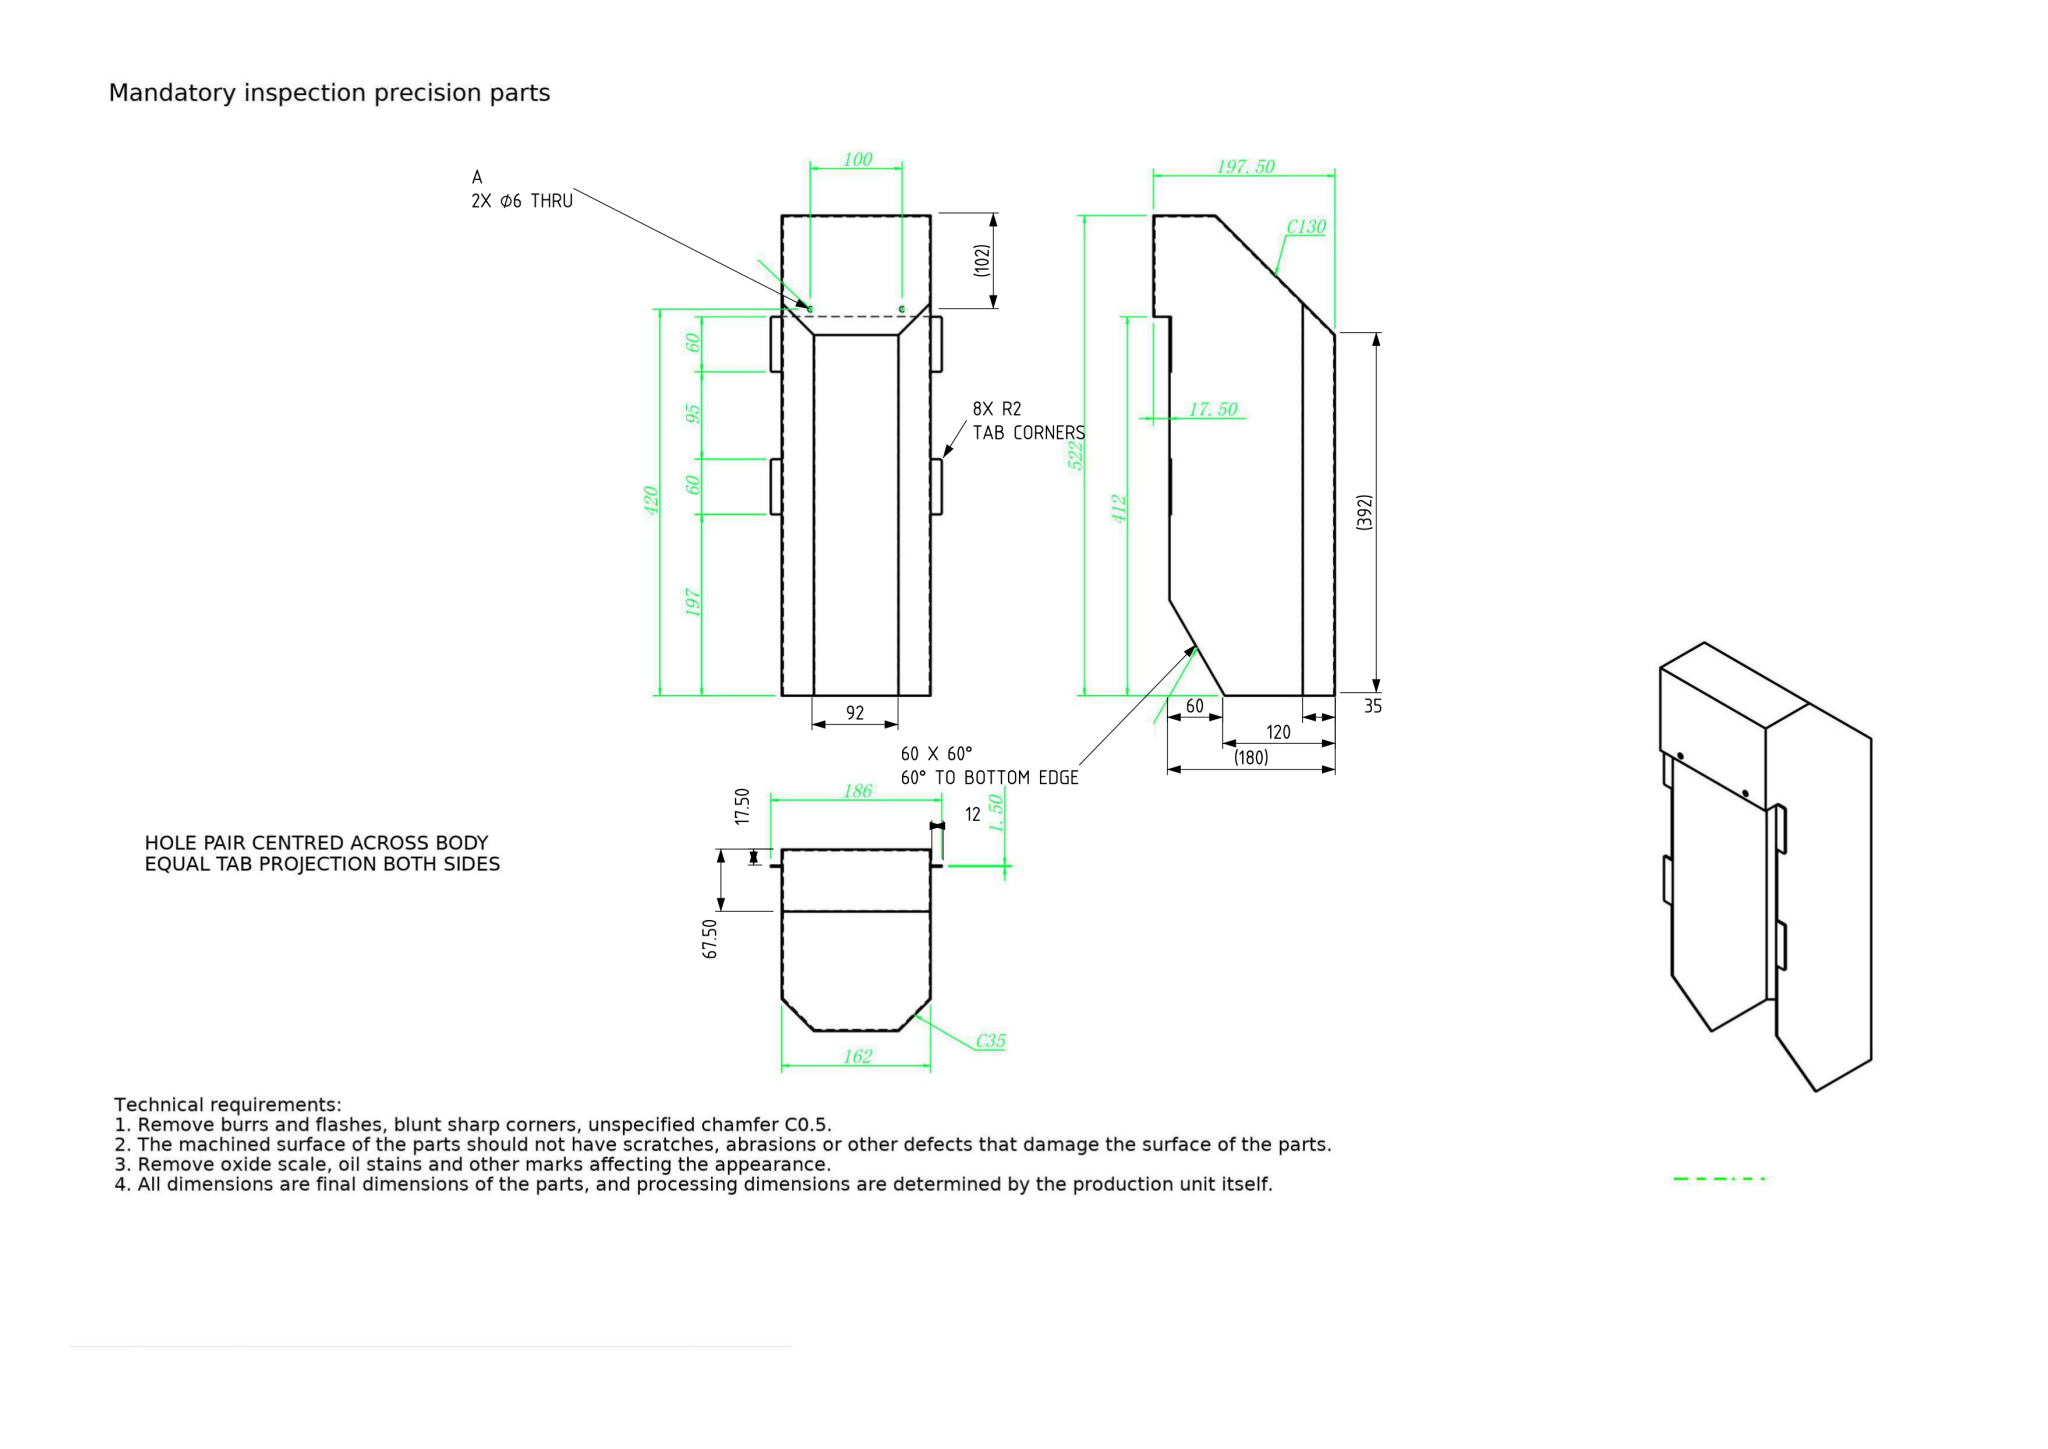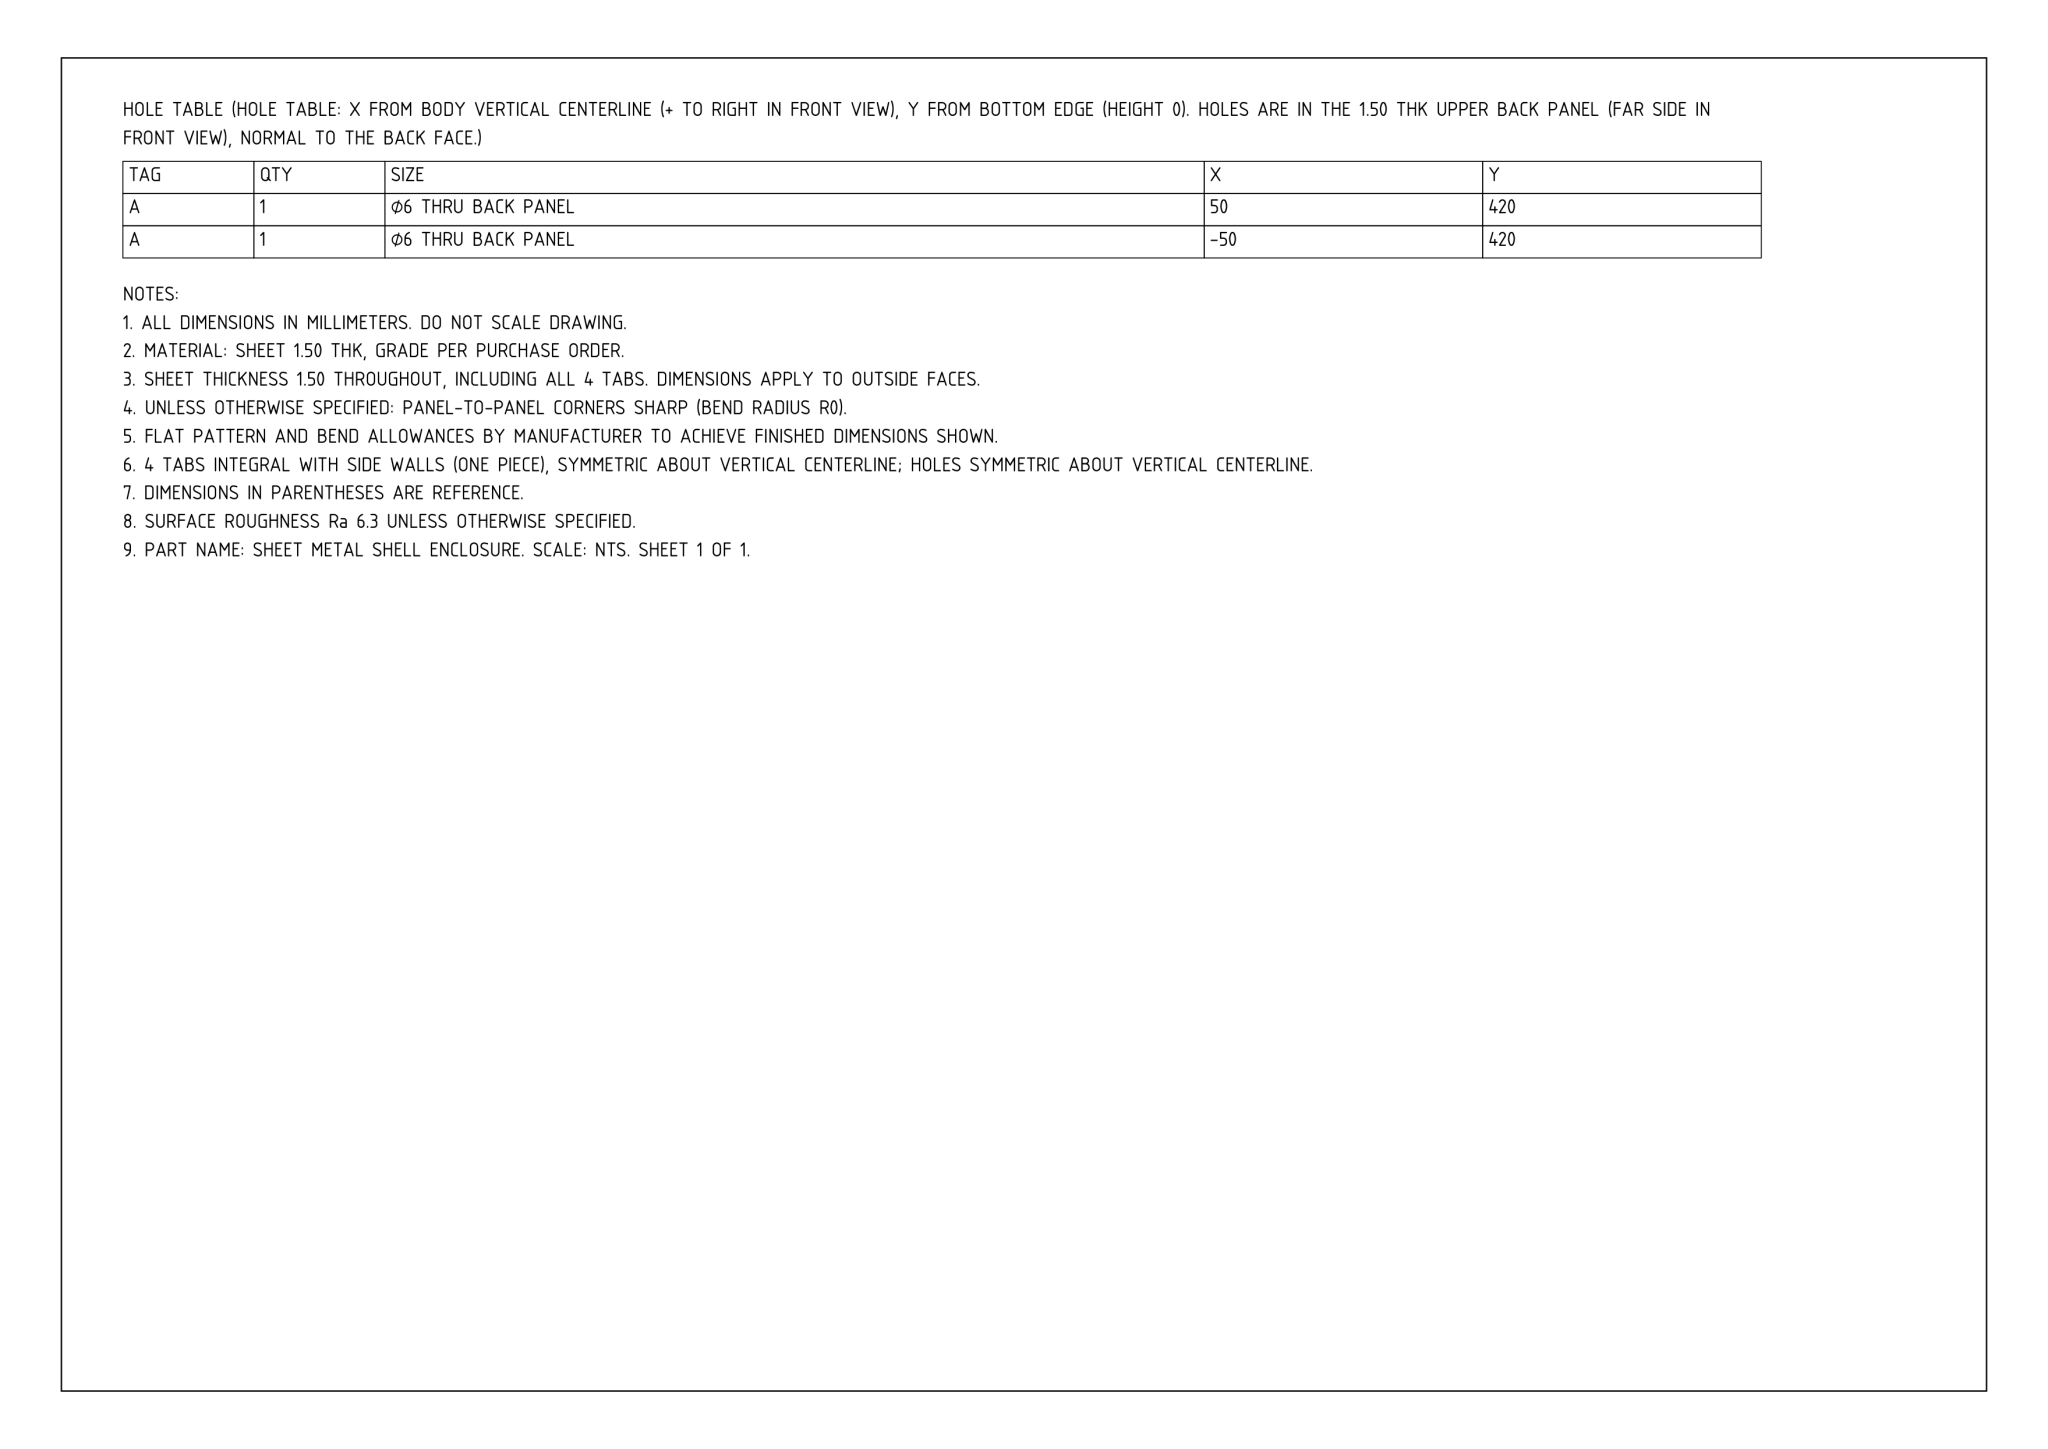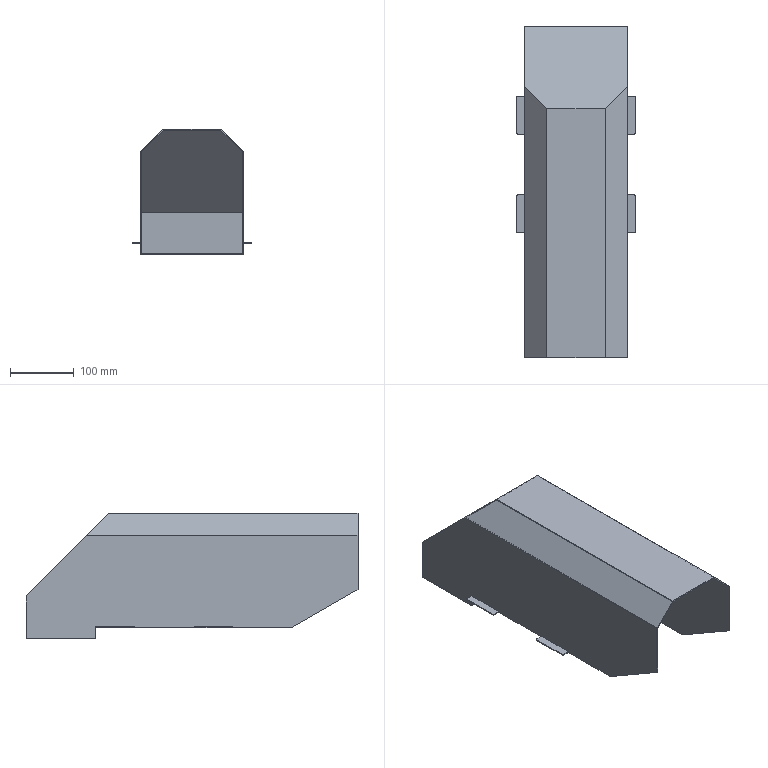Part | NX | mm | 1 solid | 50 faces | box 186 x 522 x 197.5 mm | volume 410615 mm3 | plane 38 | cylinder 12 | commonest cylinder face diameters 4 x8 6 x4